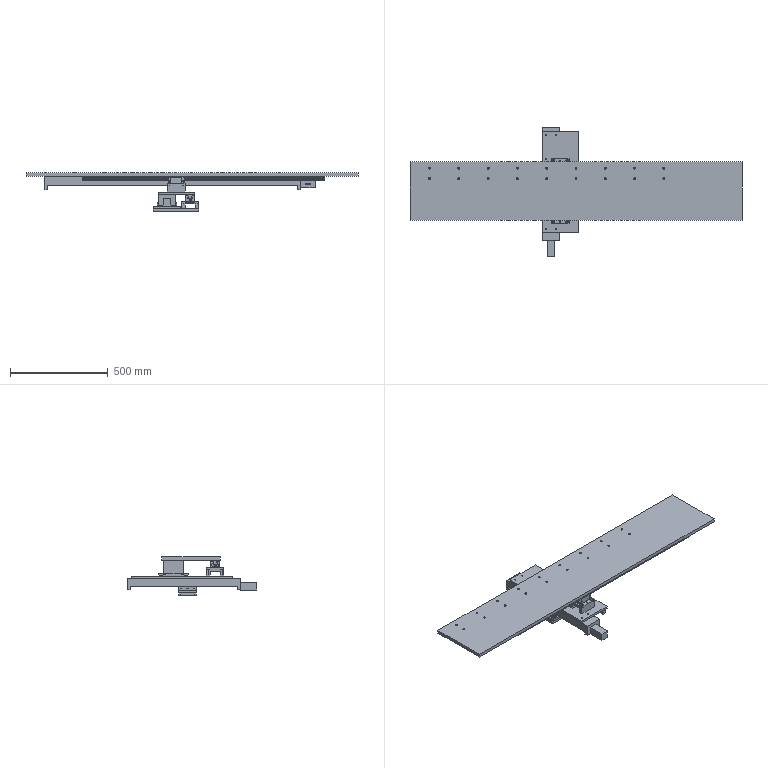Assembly | SolidWorks | mm | 17 component files | 17 solids | 2214 faces | box 1700 x 662.4 x 196.5 mm | volume 16569751 mm3 | plane 1140 | cylinder 462 | cone 316 | spline 296 | commonest cylinder face diameters 6 x72 5 x44 6.8 x40 10 x38 5.5 x36 15 x32 9 x32 11 x32
Bill of materials:
200WServoMotor | 1 |  | Rectangular block with one plain cylindrical pin or boss sticking out of one end face, and a short line of raised characters on one long side face.
GuideRailHGH25 | 1 |  | Very long straight prismatic bar with a constant, symmetric shaped cross-section. Along the top it has chamfered corners and two small chamfered notches. Below that it has angled flanks leading to a narrower waist, and the lower corners have concave rounded recesses.
GuideRailHGH25-2 | 1 |  | Straight prismatic bar with the same symmetric profile as unnamed part 1: notched and chamfered top, tapered flanks to a waist, and concave rounded recesses near the lower corners. It is shorter relative to its cross-section.
SliderHGH25 | 2 | Q235-B | Rectangular block with a lengthwise channel open on one face. The channel walls have rounded lobes and chamfered entry corners. The outer corners are chamfered, and a separate end section or plate is visible at one end. There are small holes on the end and side faces.
U-AxisSlideMountingPlate | 1 | Aluminum 6061 (GB) | Flat rectangular plate of constant thickness with about 17 through holes. There is one larger hole and many smaller holes of two apparent sizes, arranged in columns across the plate.
X-AxisSlide | 1 |  | Long rectangular bar with short downward lips at both ends, giving a very shallow inverted-channel side profile. A round hole is visible on one end face, and two rows of small holes run along the top face.
X-AxisSlideMountingPlate | 1 | Aluminum 6061 (GB) | Thin, long, flat rectangular plate with two parallel rows of small holes. The holes sit along one long edge and cover most of the plate's length, but not all of it.
X-AxisSlider | 1 |  | Solid rectangular block sitting on a wider base. The base has two downward legs along opposite edges, which form an open slot or bridge underneath.
X-AxisSliderRiserBlock | 1 | Aluminum 6061 (GB) | Nearly square block with a large rectangular slot through the underside, giving an inverted U or bridge cross-section. The top face has four large counterbored corner holes and six smaller holes. A shallow step or groove runs across the top face.
X-AxisSliderShimPlate | 1 | Aluminum 6061 (GB) | Rectangular flat plate of moderate thickness with four large counterbored holes at the corners and eight smaller through holes. The holes are arranged symmetrically in rows near each short end.
100WServoMotor | 1 |  | Rectangular block with a slender cylindrical pin sticking out of one end face. The pin is set off-centre toward one side. Small relief features appear along one face edge.
Y-AxisSlide | 1 |  | Long rectangular bar with short downward lips at both ends, giving a shallow inverted-channel profile. One end face has a round hole, and the top face has four pairs of small holes spaced along its length.
Y-AxisSlider | 1 |  | Prismatic part: a rectangular block sits centered on a wider, thinner flange. Two legs drop down at the outer ends of the flange, so the end profile is an inverted U with a raised center block.
Y-AxisSlideMountingPlate | 1 |  | Thin, elongated rectangular flat plate with a pattern of small through holes in two apparent sizes, arranged in groups along its length.
Y-AxisSliderRiserBlock | 1 | Aluminum 6061 (GB) | Rectangular block with a through channel cut into its underside, giving a bridge or inverted-U profile: two thick end walls joined by a thinner top web. The top has four large corner holes, probably counterbored, and six smaller through holes. There is a shallow step or groove on the upper surface.
Y-AxisSliderShimPlate | 1 | Aluminum 6061 (GB) | Rectangular flat plate of moderate thickness with four large corner holes, probably counterbored, and eight smaller through holes placed symmetrically near the two short ends.
Mates:
1. coincident | X-AxisSlide-1 face at (0, 0, 59) dir (0, 0, -1) | X-AxisSlider-1 face at (64.229, 35, 59) dir (0, 0, 1)
2. coincident | X-AxisSlide-1 face at (640, 35, 59) dir (0, -1, 0) | X-AxisSlider-1 face at (64.229, 35, 59) dir (0, 1, 0)
3. distance | X-AxisSlider-1 face at (64.229, 0, 59) dir (1, 0, 0) | X-AxisSlide-1 face at (640, 35, 59) dir (-1, 0, 0)
4. coincident | X-AxisSlide-1 face at (655, 50, 69) dir (1, 0, 0) | 200WServoMotor-1 face at (655, 0, 29) dir (-1, 0, 0)
5. concentric | X-AxisSlide-1 face at (633, 0, 29) dir (1, 0, 0) r 15 | 200WServoMotor-1 face at (625, 0, 29) dir (1, 0, 0) r 7
6. parallel | X-AxisSlide-1 face at (0, 0, 0) dir (0, 0, -1) | 200WServoMotor-1 face at (731.6, -20, 9) dir (0, 0, -1)
7. coincident | X-AxisSlide-1 face at (0, 0, 69) dir (0, 0, 1) | X-AxisSlideMountingPlate-1 face at (100, -90, 69) dir (0, 0, -1)
8. concentric | X-AxisSlide-1 face at (550, 27, 69) dir (0, 0, 1) r 2.1 | X-AxisSlideMountingPlate-1 face at (550, 27, 86) dir (0, 0, 1) r 2.75
9. parallel | X-AxisSlide-1 face at (-655, 50, 69) dir (0, 1, 0) | X-AxisSlideMountingPlate-1 face at (-750, 60, 86) dir (0, 1, 0)
10. coincident | X-AxisSlideMountingPlate-1 face at (100, -90, 69) dir (0, 0, -1) | GuideRailHGH25-1 face at (780, -208.571, 69) dir (0, 0, 1)
11. distance | GuideRailHGH25-1 face at (780, -202.505, 47.505) dir (1, 0, 0) | X-AxisSlideMountingPlate-1 face at (950, 60, 86) dir (1, 0, 0)
12. coincident | GuideRailHGH25-1 face at (780, -202, 50.45) dir (0, 1, 0) | SliderHGH25-1 face at (-19.271, -202, 69) dir (0, -1, 0)
13. coincident | GuideRailHGH25-1 face at (780, -221.55, 47) dir (0, 0, -1) | SliderHGH25-1 face at (-19.271, -202, 47) dir (0, 0, 1)
14. coincident | SliderHGH25-1 face at (107.342, -189.5, 29) dir (0, 0, -1) | X-AxisSliderRiserBlock-1 face at (19.229, -213.5, 29) dir (0, 0, 1)
15. coincident | SliderHGH25-1 face at (107.342, -189.5, 29) dir (0, 1, 0) | X-AxisSliderRiserBlock-1 face at (64.229, -189.5, 29) dir (0, -1, 0)
16. parallel | SliderHGH25-1 face at (36.729, -231, 29) dir (0, 0, -1) r 3 | X-AxisSliderRiserBlock-1 face at (36.729, -231, 12.5) dir (0, 0, -1) r 3.3
17. concentric | SliderHGH25-1 face at (36.729, -231, 29) dir (0, 0, -1) r 3 | X-AxisSliderRiserBlock-1 face at (36.729, -231, 12.5) dir (0, 0, -1) r 3.3
18. parallel | Y-AxisSlideMountingPlate-1 face at (111.729, 216.5, -24.5) dir (1, 0, 0) | X-AxisSliderRiserBlock-1 face at (64.229, -258.5, 31.5) dir (1, 0, 0)
19. concentric | Y-AxisSlideMountingPlate-1 face at (-15.771, -248.5, -12.5) dir (0, 0, 1) r 3.4 | X-AxisSliderRiserBlock-1 face at (-15.771, -248.5, 31.5) dir (0, 0, 1) r 4.5
20. coincident | X-AxisSlider-1 face at (64.229, -52, -0.5) dir (0, 0, -1) | X-AxisSliderShimPlate-1 face at (19.229, 0, -0.5) dir (0, 0, 1)
21. concentric | X-AxisSlider-1 face at (56.229, 47.5, 9.5) dir (0, 0, -1) r 2.5 | X-AxisSliderShimPlate-1 face at (56.229, 47.5, -12.5) dir (0, 0, -1) r 5.5
22. concentric | X-AxisSlider-1 face at (56.229, -47.5, 9.5) dir (0, 0, -1) r 2.5 | X-AxisSliderShimPlate-1 face at (56.229, -47.5, -12.5) dir (0, 0, -1) r 3.3
23. coincident | Y-AxisSlideMountingPlate-1 face at (19.229, -43.5, -12.5) dir (0, 0, 1) | X-AxisSliderShimPlate-1 face at (19.229, 0, -12.5) dir (0, 0, -1)
24. concentric | Y-AxisSlideMountingPlate-1 face at (56.229, 65, -12.5) dir (0, 0, 1) r 3.4 | X-AxisSliderShimPlate-1 face at (56.229, 65, -0.5) dir (0, 0, 1) r 7.5
25. coincident | Y-AxisSlideMountingPlate-1 face at (19.229, -43.5, -24.5) dir (0, 0, -1) | GuideRailHGH25-2-1 face at (98.944, 216.5, -24.5) dir (0, 0, 1)
26. coincident | Y-AxisSlideMountingPlate-1 face at (-73.271, 216.5, -24.5) dir (0, 1, 0) | GuideRailHGH25-2-1 face at (79.735, 216.5, -45.995) dir (0, 1, 0)
27. coincident | GuideRailHGH25-2-1 face at (98.779, 216.5, -46.5) dir (0, 0, -1) | SliderHGH25-2 face at (102.229, -33.382, -46.5) dir (0, 0, 1)
28. coincident | GuideRailHGH25-2-1 face at (102.229, 216.5, -39.9) dir (1, 0, 0) | SliderHGH25-2 face at (102.229, -33.382, -24.5) dir (-1, 0, 0)
29. coincident | SliderHGH25-2 face at (114.729, -159.994, -64.5) dir (0, 0, -1) | Y-AxisSliderRiserBlock-1 face at (90.729, -71.882, -64.5) dir (0, 0, 1)
30. coincident | SliderHGH25-2 face at (114.729, -159.994, -64.5) dir (1, 0, 0) | Y-AxisSliderRiserBlock-1 face at (114.729, -26.882, -64.5) dir (-1, 0, 0)
31. concentric | SliderHGH25-2 face at (108.229, -54.382, -64.5) dir (0, 0, -1) r 3 | Y-AxisSliderRiserBlock-1 face at (108.229, -54.382, -73.5) dir (0, 0, -1) r 3.3
32. coincident | Y-AxisAssembly-1/Y-AxisSlide-1 face at (-28.271, -53.5, -24.5) dir (0, 0, 1) | Y-AxisSlideMountingPlate-1 face at (19.229, -43.5, -24.5) dir (0, 0, -1)
33. concentric | Y-AxisAssembly-1/Y-AxisSlide-1 face at (-53.271, -283.5, -2.5) dir (0, 0, -1) r 3.5 | Y-AxisSlideMountingPlate-1 face at (-53.271, -283.5, -24.5) dir (0, 0, -1) r 2.5
34. concentric | Y-AxisAssembly-1/Y-AxisSlide-1 face at (-3.271, -283.5, -2.5) dir (0, 0, -1) r 3.5 | Y-AxisSlideMountingPlate-1 face at (-3.271, -283.5, -24.5) dir (0, 0, -1) r 2.5
35. concentric | Y-AxisAssembly-1/Y-AxisSlider-1 face at (16.729, -106.882, -76.5) dir (0, 0, -1) r 3 | Y-AxisSliderShimPlate-1 face at (16.729, -106.882, -98.5) dir (0, 0, -1) r 3.3
36. concentric | Y-AxisAssembly-1/Y-AxisSlider-1 face at (16.729, -36.882, -76.5) dir (0, 0, -1) r 3 | Y-AxisSliderShimPlate-1 face at (16.729, -36.882, -98.5) dir (0, 0, -1) r 5.5
37. coincident | Y-AxisAssembly-1/Y-AxisSlider-1 face at (21.729, -116.882, -86.5) dir (0, 0, -1) | Y-AxisSliderShimPlate-1 face at (-28.271, -71.882, -86.5) dir (0, 0, 1)
38. parallel | U-AxisSlideMountingPlate-1 face at (135.729, -26.882, -98.5) dir (0, 1, 0) | Y-AxisSliderRiserBlock-1 face at (135.729, -26.882, -62) dir (0, 1, 0)
39. concentric | U-AxisSlideMountingPlate-1 face at (125.729, -36.882, -98.5) dir (0, 0, 1) r 3.4 | Y-AxisSliderRiserBlock-1 face at (125.729, -36.882, -62) dir (0, 0, 1) r 4.5
40. coincident | U-AxisSlideMountingPlate-1 face at (18.729, -71.882, -98.5) dir (0, 0, 1) | Y-AxisSliderShimPlate-1 face at (-28.271, -71.882, -98.5) dir (0, 0, -1)
41. concentric | U-AxisSlideMountingPlate-1 face at (31.729, -36.882, -98.5) dir (0, 0, 1) r 3.4 | Y-AxisSliderShimPlate-1 face at (31.729, -36.882, -86.5) dir (0, 0, 1) r 4.5
42. coincident | Y-AxisSlide-1 face at (0, 0, 48) dir (0, 0, -1) | Y-AxisSlider-1 face at (63.382, -30, 48) dir (0, 0, 1)
43. coincident | Y-AxisSlide-1 face at (271.976, -30, 48) dir (0, 1, 0) | Y-AxisSlider-1 face at (63.382, -30, 16) dir (0, -1, 0)
44. distance | Y-AxisSlider-1 face at (-26.618, 0, 28.6) dir (-1, 0, 0) | Y-AxisSlide-1 face at (271.976, 30, 48) dir (-1, 0, 0)
45. coincident | Y-AxisSlide-1 face at (290, 45, 58) dir (1, 0, 0) | 100WServoMotor-1 face at (290, 0, 18) dir (-1, 0, 0)
46. concentric | Y-AxisSlide-1 face at (260, 0, 18) dir (1, 0, 0) r 17 | 100WServoMotor-1 face at (260, 0, 18) dir (1, 0, 0) r 4
47. parallel | Y-AxisSlide-1 face at (0, 0, 0) dir (0, 0, -1) | 100WServoMotor-1 face at (372.4, 20, -2) dir (0, 0, -1)